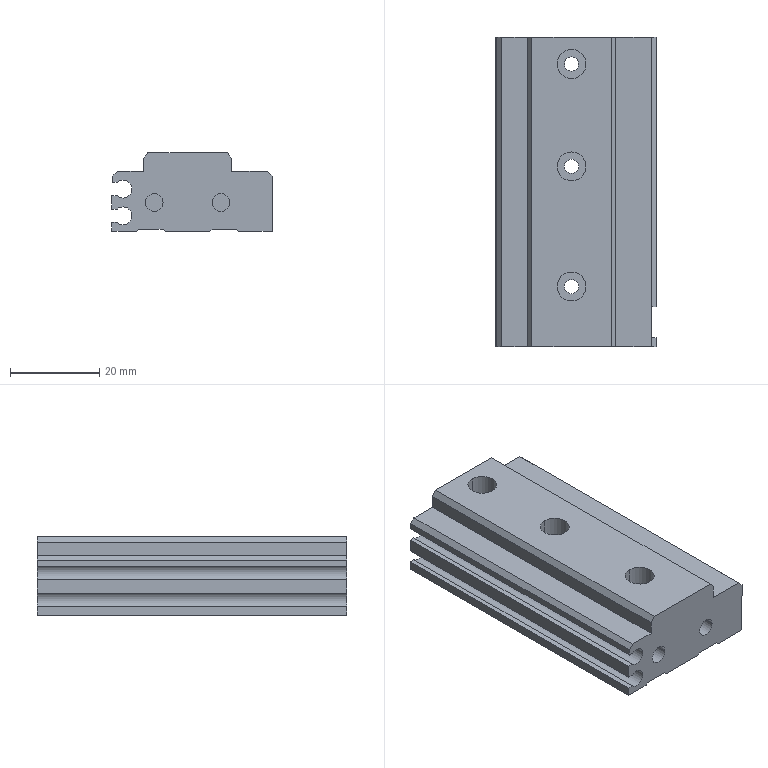Component | SolidWorks | MXQ8L-30B-M9N_0_0_MXQ8L-30B-M9N_0_0-1_MXQ8L-30B-M9N_0_0_1_27-1 | 1 solid | 133 faces | volume 31535 mm3 | plane 58 | cylinder 57 | cone 18 | commonest cylinder face diameters 2.459 x12 6.5 x6 4 x6 3.2 x6 3.242 x6 3 x5 4.134 x4 5 x4